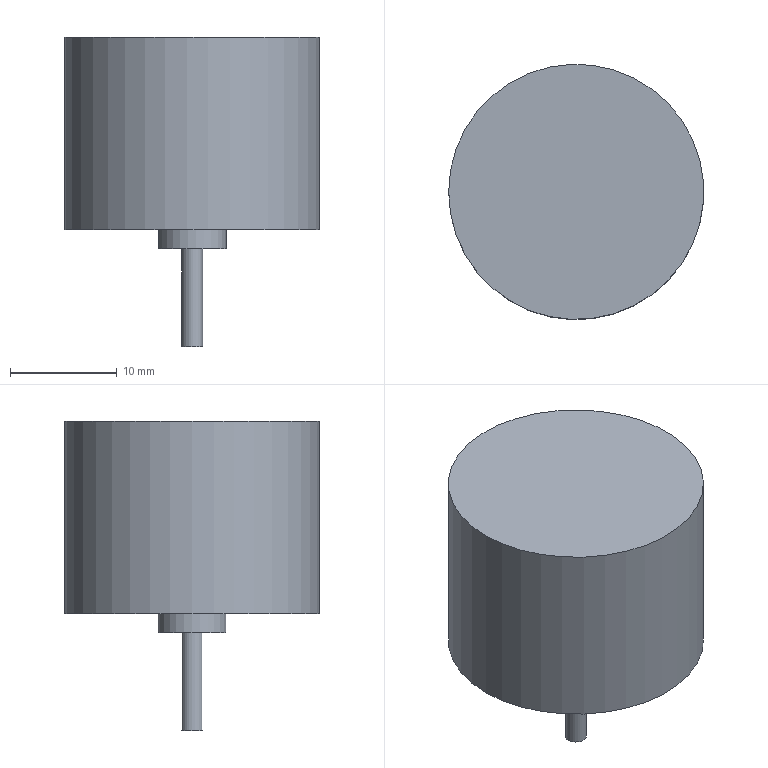Component | NX | MOTOR | 1 solid | 7 faces | box 23.9 x 23.9 x 28.95 mm | volume 8160 mm3 | plane 4 | cylinder 3 | commonest cylinder face diameters 23.9 x1 6.34 x1 1.96 x1
STEP:
#1=CARTESIAN_POINT('',(0.,0.,0.));
#2=DIRECTION('',(0.,0.,1.));
#3=DIRECTION('',(1.,0.,0.));
#4=AXIS2_PLACEMENT_3D('',#1,#2,#3);
#5=CARTESIAN_POINT('',(-2.325,0.6765,-8.224));
#6=VERTEX_POINT('',#5);
#7=CARTESIAN_POINT('',(0.8451,0.6765,-8.224));
#8=DIRECTION('',(0.,0.,-1.));
#9=DIRECTION('',(-1.,0.,0.));
#10=AXIS2_PLACEMENT_3D('',#7,#8,#9);
#11=CIRCLE('',#10,3.17);
#12=CARTESIAN_POINT('',(0.8451,0.6765,-8.224));
#13=DIRECTION('',(0.,0.,-1.));
#14=DIRECTION('',(-1.,0.,0.));
#15=AXIS2_PLACEMENT_3D('',#12,#13,#14);
#16=PLANE('',#15);
#17=CARTESIAN_POINT('',(0.,0.));
#18=DIRECTION('',(1.,0.));
#19=AXIS2_PLACEMENT_2D('',#17,#18);
#20=CIRCLE('',#19,3.17);
#21=(GEOMETRIC_REPRESENTATION_CONTEXT(2)PARAMETRIC_REPRESENTATION_CONTEXT()REPRESENTATION_CONTEXT('',''));
#22=DEFINITIONAL_REPRESENTATION('',(#20),#21);
#23=PCURVE('',#16,#22);
#24=CARTESIAN_POINT('',(0.8451,0.6765,-8.224));
#25=DIRECTION('',(0.,0.,-1.));
#26=DIRECTION('',(-1.,0.,0.));
#27=AXIS2_PLACEMENT_3D('',#24,#25,#26);
#28=CYLINDRICAL_SURFACE('',#27,3.17);
#29=CARTESIAN_POINT('',(0.,0.));
#30=DIRECTION('',(1.,0.));
#31=VECTOR('',#30,1.);
#32=LINE('',#29,#31);
#33=(GEOMETRIC_REPRESENTATION_CONTEXT(2)PARAMETRIC_REPRESENTATION_CONTEXT()REPRESENTATION_CONTEXT('',''));
#34=DEFINITIONAL_REPRESENTATION('',(#32),#33);
#35=PCURVE('',#28,#34);
#36=SURFACE_CURVE('',#11,(#23,#35),.PCURVE_S1.);
#37=EDGE_CURVE('',#6,#6,#36,.T.);
#38=ORIENTED_EDGE('',*,*,#37,.F.);
#39=EDGE_LOOP('',(#38));
#40=FACE_BOUND('',#39,.T.);
#41=CARTESIAN_POINT('',(-11.105,0.6765,-8.224));
#42=VERTEX_POINT('',#41);
#43=CARTESIAN_POINT('',(0.8451,0.6765,-8.224));
#44=DIRECTION('',(0.,0.,1.));
#45=DIRECTION('',(-1.,0.,0.));
#46=AXIS2_PLACEMENT_3D('',#43,#44,#45);
#47=CIRCLE('',#46,11.95);
#48=CARTESIAN_POINT('',(11.95,0.));
#49=CARTESIAN_POINT('',(11.95,-20.698));
#50=CARTESIAN_POINT('',(-5.975,-10.349));
#51=CARTESIAN_POINT('',(-23.9,-0.));
#52=CARTESIAN_POINT('',(-5.975,10.349));
#53=CARTESIAN_POINT('',(11.95,20.698));
#54=CARTESIAN_POINT('',(11.95,0.));
#55=(BOUNDED_CURVE()B_SPLINE_CURVE(2,(#48,#49,#50,#51,#52,#53,#54),.UNSPECIFIED.,.T.,.F.)B_SPLINE_CURVE_WITH_KNOTS((1,2,2,2,2,1),(-2.094,0.,2.094,4.189,6.283,8.378),.UNSPECIFIED.)CURVE()GEOMETRIC_REPRESENTATION_ITEM()RATIONAL_B_SPLINE_CURVE((1.,0.5,1.,0.5,1.,0.5,1.))REPRESENTATION_ITEM(''));
#56=(GEOMETRIC_REPRESENTATION_CONTEXT(2)PARAMETRIC_REPRESENTATION_CONTEXT()REPRESENTATION_CONTEXT('',''));
#57=DEFINITIONAL_REPRESENTATION('',(#55),#56);
#58=PCURVE('',#16,#57);
#59=CARTESIAN_POINT('',(0.8451,0.6765,9.776));
#60=DIRECTION('',(0.,0.,-1.));
#61=DIRECTION('',(-1.,0.,0.));
#62=AXIS2_PLACEMENT_3D('',#59,#60,#61);
#63=CYLINDRICAL_SURFACE('',#62,11.95);
#64=CARTESIAN_POINT('',(6.283,18.));
#65=DIRECTION('',(-1.,0.));
#66=VECTOR('',#65,1.);
#67=LINE('',#64,#66);
#68=(GEOMETRIC_REPRESENTATION_CONTEXT(2)PARAMETRIC_REPRESENTATION_CONTEXT()REPRESENTATION_CONTEXT('',''));
#69=DEFINITIONAL_REPRESENTATION('',(#67),#68);
#70=PCURVE('',#63,#69);
#71=SURFACE_CURVE('',#47,(#58,#70),.PCURVE_S1.);
#72=EDGE_CURVE('',#42,#42,#71,.T.);
#73=ORIENTED_EDGE('',*,*,#72,.F.);
#74=EDGE_LOOP('',(#73));
#75=FACE_BOUND('',#74,.T.);
#76=ADVANCED_FACE('',(#40,#75),#16,.T.);
#77=CARTESIAN_POINT('',(-11.105,0.6765,9.776));
#78=VERTEX_POINT('',#77);
#79=CARTESIAN_POINT('',(0.8451,0.6765,9.776));
#80=DIRECTION('',(0.,0.,-1.));
#81=DIRECTION('',(-1.,0.,0.));
#82=AXIS2_PLACEMENT_3D('',#79,#80,#81);
#83=CIRCLE('',#82,11.95);
#84=CARTESIAN_POINT('',(0.8451,0.6765,9.776));
#85=DIRECTION('',(0.,0.,1.));
#86=DIRECTION('',(1.,0.,0.));
#87=AXIS2_PLACEMENT_3D('',#84,#85,#86);
#88=PLANE('',#87);
#89=CARTESIAN_POINT('',(-11.95,0.));
#90=CARTESIAN_POINT('',(-11.95,20.698));
#91=CARTESIAN_POINT('',(5.975,10.349));
#92=CARTESIAN_POINT('',(23.9,0.));
#93=CARTESIAN_POINT('',(5.975,-10.349));
#94=CARTESIAN_POINT('',(-11.95,-20.698));
#95=CARTESIAN_POINT('',(-11.95,0.));
#96=(BOUNDED_CURVE()B_SPLINE_CURVE(2,(#89,#90,#91,#92,#93,#94,#95),.UNSPECIFIED.,.T.,.F.)B_SPLINE_CURVE_WITH_KNOTS((1,2,2,2,2,1),(-2.094,0.,2.094,4.189,6.283,8.378),.UNSPECIFIED.)CURVE()GEOMETRIC_REPRESENTATION_ITEM()RATIONAL_B_SPLINE_CURVE((1.,0.5,1.,0.5,1.,0.5,1.))REPRESENTATION_ITEM(''));
#97=(GEOMETRIC_REPRESENTATION_CONTEXT(2)PARAMETRIC_REPRESENTATION_CONTEXT()REPRESENTATION_CONTEXT('',''));
#98=DEFINITIONAL_REPRESENTATION('',(#96),#97);
#99=PCURVE('',#88,#98);
#100=CARTESIAN_POINT('',(0.,0.));
#101=DIRECTION('',(1.,0.));
#102=VECTOR('',#101,1.);
#103=LINE('',#100,#102);
#104=(GEOMETRIC_REPRESENTATION_CONTEXT(2)PARAMETRIC_REPRESENTATION_CONTEXT()REPRESENTATION_CONTEXT('',''));
#105=DEFINITIONAL_REPRESENTATION('',(#103),#104);
#106=PCURVE('',#63,#105);
#107=SURFACE_CURVE('',#83,(#99,#106),.PCURVE_S1.);
#108=EDGE_CURVE('',#78,#78,#107,.T.);
#109=ORIENTED_EDGE('',*,*,#108,.F.);
#110=EDGE_LOOP('',(#109));
#111=FACE_BOUND('',#110,.T.);
#112=ADVANCED_FACE('',(#111),#88,.T.);
#113=ORIENTED_EDGE('',*,*,#72,.T.);
#114=CARTESIAN_POINT('',(-11.105,0.6765,9.776));
#115=CARTESIAN_POINT('',(-11.105,0.6765,-8.224));
#116=B_SPLINE_CURVE_WITH_KNOTS('',1,(#114,#115),.UNSPECIFIED.,.F.,.F.,(2,2),(0.,18.),.PIECEWISE_BEZIER_KNOTS.);
#117=CARTESIAN_POINT('',(0.,0.));
#118=DIRECTION('',(0.,1.));
#119=VECTOR('',#118,1.);
#120=LINE('',#117,#119);
#121=(GEOMETRIC_REPRESENTATION_CONTEXT(2)PARAMETRIC_REPRESENTATION_CONTEXT()REPRESENTATION_CONTEXT('',''));
#122=DEFINITIONAL_REPRESENTATION('',(#120),#121);
#123=PCURVE('',#63,#122);
#124=CARTESIAN_POINT('',(6.283,0.));
#125=DIRECTION('',(0.,1.));
#126=VECTOR('',#125,1.);
#127=LINE('',#124,#126);
#128=(GEOMETRIC_REPRESENTATION_CONTEXT(2)PARAMETRIC_REPRESENTATION_CONTEXT()REPRESENTATION_CONTEXT('',''));
#129=DEFINITIONAL_REPRESENTATION('',(#127),#128);
#130=PCURVE('',#63,#129);
#131=SEAM_CURVE('',#116,(#123,#130),.PCURVE_S1.);
#132=EDGE_CURVE('',#78,#42,#131,.T.);
#133=ORIENTED_EDGE('',*,*,#132,.F.);
#134=ORIENTED_EDGE('',*,*,#108,.T.);
#135=ORIENTED_EDGE('',*,*,#132,.T.);
#136=EDGE_LOOP('',(#113,#133,#134,#135));
#137=FACE_BOUND('',#136,.T.);
#138=ADVANCED_FACE('',(#137),#63,.T.);
#139=CARTESIAN_POINT('',(-0.1349,0.6765,-10.024));
#140=VERTEX_POINT('',#139);
#141=CARTESIAN_POINT('',(0.8451,0.6765,-10.024));
#142=DIRECTION('',(0.,0.,-1.));
#143=DIRECTION('',(-1.,0.,0.));
#144=AXIS2_PLACEMENT_3D('',#141,#142,#143);
#145=CIRCLE('',#144,0.98);
#146=CARTESIAN_POINT('',(0.8451,0.6765,-10.024));
#147=DIRECTION('',(0.,0.,-1.));
#148=DIRECTION('',(-1.,0.,0.));
#149=AXIS2_PLACEMENT_3D('',#146,#147,#148);
#150=PLANE('',#149);
#151=CARTESIAN_POINT('',(0.,0.));
#152=DIRECTION('',(1.,0.));
#153=AXIS2_PLACEMENT_2D('',#151,#152);
#154=CIRCLE('',#153,0.98);
#155=(GEOMETRIC_REPRESENTATION_CONTEXT(2)PARAMETRIC_REPRESENTATION_CONTEXT()REPRESENTATION_CONTEXT('',''));
#156=DEFINITIONAL_REPRESENTATION('',(#154),#155);
#157=PCURVE('',#150,#156);
#158=CARTESIAN_POINT('',(0.8451,0.6765,-10.024));
#159=DIRECTION('',(0.,0.,-1.));
#160=DIRECTION('',(-1.,0.,0.));
#161=AXIS2_PLACEMENT_3D('',#158,#159,#160);
#162=CYLINDRICAL_SURFACE('',#161,0.98);
#163=CARTESIAN_POINT('',(0.,0.));
#164=DIRECTION('',(1.,0.));
#165=VECTOR('',#164,1.);
#166=LINE('',#163,#165);
#167=(GEOMETRIC_REPRESENTATION_CONTEXT(2)PARAMETRIC_REPRESENTATION_CONTEXT()REPRESENTATION_CONTEXT('',''));
#168=DEFINITIONAL_REPRESENTATION('',(#166),#167);
#169=PCURVE('',#162,#168);
#170=SURFACE_CURVE('',#145,(#157,#169),.PCURVE_S1.);
#171=EDGE_CURVE('',#140,#140,#170,.T.);
#172=ORIENTED_EDGE('',*,*,#171,.F.);
#173=EDGE_LOOP('',(#172));
#174=FACE_BOUND('',#173,.T.);
#175=CARTESIAN_POINT('',(-2.325,0.6765,-10.024));
#176=VERTEX_POINT('',#175);
#177=CARTESIAN_POINT('',(0.8451,0.6765,-10.024));
#178=DIRECTION('',(0.,0.,1.));
#179=DIRECTION('',(-1.,0.,0.));
#180=AXIS2_PLACEMENT_3D('',#177,#178,#179);
#181=CIRCLE('',#180,3.17);
#182=CARTESIAN_POINT('',(3.17,0.));
#183=CARTESIAN_POINT('',(3.17,-5.491));
#184=CARTESIAN_POINT('',(-1.585,-2.745));
#185=CARTESIAN_POINT('',(-6.34,-0.));
#186=CARTESIAN_POINT('',(-1.585,2.745));
#187=CARTESIAN_POINT('',(3.17,5.491));
#188=CARTESIAN_POINT('',(3.17,0.));
#189=(BOUNDED_CURVE()B_SPLINE_CURVE(2,(#182,#183,#184,#185,#186,#187,#188),.UNSPECIFIED.,.T.,.F.)B_SPLINE_CURVE_WITH_KNOTS((1,2,2,2,2,1),(-2.094,0.,2.094,4.189,6.283,8.378),.UNSPECIFIED.)CURVE()GEOMETRIC_REPRESENTATION_ITEM()RATIONAL_B_SPLINE_CURVE((1.,0.5,1.,0.5,1.,0.5,1.))REPRESENTATION_ITEM(''));
#190=(GEOMETRIC_REPRESENTATION_CONTEXT(2)PARAMETRIC_REPRESENTATION_CONTEXT()REPRESENTATION_CONTEXT('',''));
#191=DEFINITIONAL_REPRESENTATION('',(#189),#190);
#192=PCURVE('',#150,#191);
#193=CARTESIAN_POINT('',(6.283,1.8));
#194=DIRECTION('',(-1.,0.));
#195=VECTOR('',#194,1.);
#196=LINE('',#193,#195);
#197=(GEOMETRIC_REPRESENTATION_CONTEXT(2)PARAMETRIC_REPRESENTATION_CONTEXT()REPRESENTATION_CONTEXT('',''));
#198=DEFINITIONAL_REPRESENTATION('',(#196),#197);
#199=PCURVE('',#28,#198);
#200=SURFACE_CURVE('',#181,(#192,#199),.PCURVE_S1.);
#201=EDGE_CURVE('',#176,#176,#200,.T.);
#202=ORIENTED_EDGE('',*,*,#201,.F.);
#203=EDGE_LOOP('',(#202));
#204=FACE_BOUND('',#203,.T.);
#205=ADVANCED_FACE('',(#174,#204),#150,.T.);
#206=ORIENTED_EDGE('',*,*,#201,.T.);
#207=CARTESIAN_POINT('',(-2.325,0.6765,-8.224));
#208=CARTESIAN_POINT('',(-2.325,0.6765,-10.024));
#209=B_SPLINE_CURVE_WITH_KNOTS('',1,(#207,#208),.UNSPECIFIED.,.F.,.F.,(2,2),(0.,1.8),.PIECEWISE_BEZIER_KNOTS.);
#210=CARTESIAN_POINT('',(0.,0.));
#211=DIRECTION('',(0.,1.));
#212=VECTOR('',#211,1.);
#213=LINE('',#210,#212);
#214=(GEOMETRIC_REPRESENTATION_CONTEXT(2)PARAMETRIC_REPRESENTATION_CONTEXT()REPRESENTATION_CONTEXT('',''));
#215=DEFINITIONAL_REPRESENTATION('',(#213),#214);
#216=PCURVE('',#28,#215);
#217=CARTESIAN_POINT('',(6.283,0.));
#218=DIRECTION('',(0.,1.));
#219=VECTOR('',#218,1.);
#220=LINE('',#217,#219);
#221=(GEOMETRIC_REPRESENTATION_CONTEXT(2)PARAMETRIC_REPRESENTATION_CONTEXT()REPRESENTATION_CONTEXT('',''));
#222=DEFINITIONAL_REPRESENTATION('',(#220),#221);
#223=PCURVE('',#28,#222);
#224=SEAM_CURVE('',#209,(#216,#223),.PCURVE_S1.);
#225=EDGE_CURVE('',#6,#176,#224,.T.);
#226=ORIENTED_EDGE('',*,*,#225,.F.);
#227=ORIENTED_EDGE('',*,*,#37,.T.);
#228=ORIENTED_EDGE('',*,*,#225,.T.);
#229=EDGE_LOOP('',(#206,#226,#227,#228));
#230=FACE_BOUND('',#229,.T.);
#231=ADVANCED_FACE('',(#230),#28,.T.);
#232=CARTESIAN_POINT('',(-0.1349,0.6765,-19.174));
#233=VERTEX_POINT('',#232);
#234=CARTESIAN_POINT('',(0.8451,0.6765,-19.174));
#235=DIRECTION('',(0.,0.,1.));
#236=DIRECTION('',(-1.,0.,0.));
#237=AXIS2_PLACEMENT_3D('',#234,#235,#236);
#238=CIRCLE('',#237,0.98);
#239=CARTESIAN_POINT('',(0.8451,0.6765,-19.174));
#240=DIRECTION('',(0.,0.,-1.));
#241=DIRECTION('',(-1.,0.,0.));
#242=AXIS2_PLACEMENT_3D('',#239,#240,#241);
#243=PLANE('',#242);
#244=CARTESIAN_POINT('',(0.98,0.));
#245=CARTESIAN_POINT('',(0.98,-1.697));
#246=CARTESIAN_POINT('',(-0.49,-0.8487));
#247=CARTESIAN_POINT('',(-1.96,-0.));
#248=CARTESIAN_POINT('',(-0.49,0.8487));
#249=CARTESIAN_POINT('',(0.98,1.697));
#250=CARTESIAN_POINT('',(0.98,0.));
#251=(BOUNDED_CURVE()B_SPLINE_CURVE(2,(#244,#245,#246,#247,#248,#249,#250),.UNSPECIFIED.,.T.,.F.)B_SPLINE_CURVE_WITH_KNOTS((1,2,2,2,2,1),(-2.094,0.,2.094,4.189,6.283,8.378),.UNSPECIFIED.)CURVE()GEOMETRIC_REPRESENTATION_ITEM()RATIONAL_B_SPLINE_CURVE((1.,0.5,1.,0.5,1.,0.5,1.))REPRESENTATION_ITEM(''));
#252=(GEOMETRIC_REPRESENTATION_CONTEXT(2)PARAMETRIC_REPRESENTATION_CONTEXT()REPRESENTATION_CONTEXT('',''));
#253=DEFINITIONAL_REPRESENTATION('',(#251),#252);
#254=PCURVE('',#243,#253);
#255=CARTESIAN_POINT('',(6.283,9.15));
#256=DIRECTION('',(-1.,0.));
#257=VECTOR('',#256,1.);
#258=LINE('',#255,#257);
#259=(GEOMETRIC_REPRESENTATION_CONTEXT(2)PARAMETRIC_REPRESENTATION_CONTEXT()REPRESENTATION_CONTEXT('',''));
#260=DEFINITIONAL_REPRESENTATION('',(#258),#259);
#261=PCURVE('',#162,#260);
#262=SURFACE_CURVE('',#238,(#254,#261),.PCURVE_S1.);
#263=EDGE_CURVE('',#233,#233,#262,.T.);
#264=ORIENTED_EDGE('',*,*,#263,.F.);
#265=EDGE_LOOP('',(#264));
#266=FACE_BOUND('',#265,.T.);
#267=ADVANCED_FACE('',(#266),#243,.T.);
#268=ORIENTED_EDGE('',*,*,#263,.T.);
#269=CARTESIAN_POINT('',(-0.1349,0.6765,-10.024));
#270=CARTESIAN_POINT('',(-0.1349,0.6765,-19.174));
#271=B_SPLINE_CURVE_WITH_KNOTS('',1,(#269,#270),.UNSPECIFIED.,.F.,.F.,(2,2),(0.,9.15),.PIECEWISE_BEZIER_KNOTS.);
#272=CARTESIAN_POINT('',(0.,0.));
#273=DIRECTION('',(0.,1.));
#274=VECTOR('',#273,1.);
#275=LINE('',#272,#274);
#276=(GEOMETRIC_REPRESENTATION_CONTEXT(2)PARAMETRIC_REPRESENTATION_CONTEXT()REPRESENTATION_CONTEXT('',''));
#277=DEFINITIONAL_REPRESENTATION('',(#275),#276);
#278=PCURVE('',#162,#277);
#279=CARTESIAN_POINT('',(6.283,0.));
#280=DIRECTION('',(0.,1.));
#281=VECTOR('',#280,1.);
#282=LINE('',#279,#281);
#283=(GEOMETRIC_REPRESENTATION_CONTEXT(2)PARAMETRIC_REPRESENTATION_CONTEXT()REPRESENTATION_CONTEXT('',''));
#284=DEFINITIONAL_REPRESENTATION('',(#282),#283);
#285=PCURVE('',#162,#284);
#286=SEAM_CURVE('',#271,(#278,#285),.PCURVE_S1.);
#287=EDGE_CURVE('',#140,#233,#286,.T.);
#288=ORIENTED_EDGE('',*,*,#287,.F.);
#289=ORIENTED_EDGE('',*,*,#171,.T.);
#290=ORIENTED_EDGE('',*,*,#287,.T.);
#291=EDGE_LOOP('',(#268,#288,#289,#290));
#292=FACE_BOUND('',#291,.T.);
#293=ADVANCED_FACE('',(#292),#162,.T.);
#294=CLOSED_SHELL('',(#76,#112,#138,#205,#231,#267,#293));
#295=MANIFOLD_SOLID_BREP('',#294);
#296=(LENGTH_UNIT()NAMED_UNIT(*)SI_UNIT(.MILLI.,.METRE.));
#297=UNCERTAINTY_MEASURE_WITH_UNIT(LENGTH_MEASURE(0.00001),#296,'','');
#298=(NAMED_UNIT(*)PLANE_ANGLE_UNIT()SI_UNIT($,.RADIAN.));
#299=(NAMED_UNIT(*)SI_UNIT($,.STERADIAN.)SOLID_ANGLE_UNIT());
#300=(GEOMETRIC_REPRESENTATION_CONTEXT(3)GLOBAL_UNCERTAINTY_ASSIGNED_CONTEXT((#297))GLOBAL_UNIT_ASSIGNED_CONTEXT((#296,#298,#299))REPRESENTATION_CONTEXT('',''));
#301=ADVANCED_BREP_SHAPE_REPRESENTATION('',(#4,#295),#300);